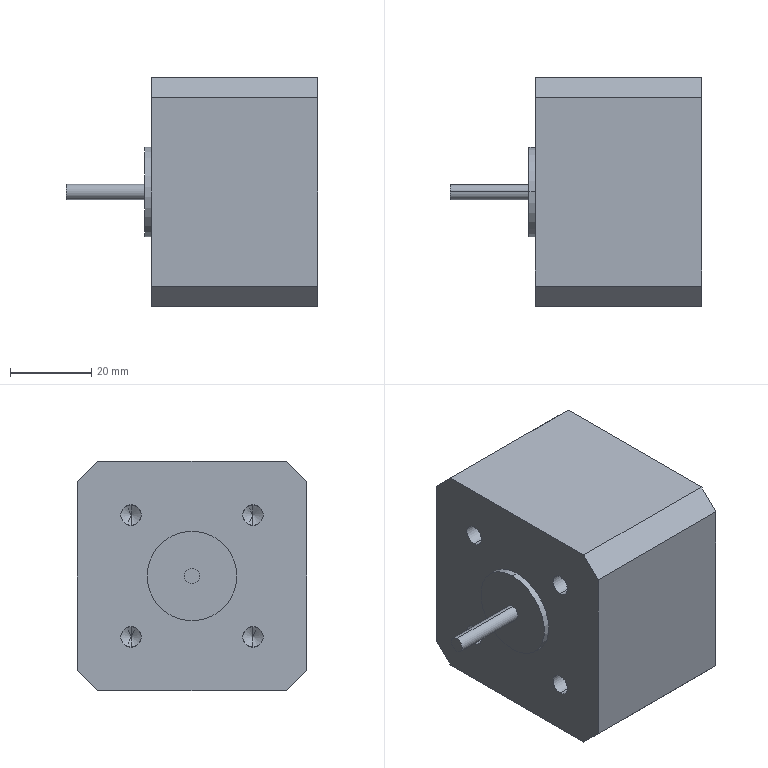Component | SolidWorks | 42StepperMotor-2 | 1 solid | 40 faces | box 62 x 56.4 x 56.4 mm | volume 128490 mm3 | cone 16 | cylinder 12 | plane 12 | commonest cylinder face diameters 5 x8 3.75 x2 22.1 x2
build123d program:
from build123d import *

# Parameters (mm, degrees)
BOSS_EXTRUDE1_DEPTH             = 41
SKETCH2_R                       = 11.05
BOSS_EXTRUDE2_DEPTH             = 1.6
SKETCH3_R                       = 1.875
BOSS_EXTRUDE3_DEPTH             = 19.4
F_5_0MM_DOWEL_HOLE1_D           = 5
F_5_0MM_DOWEL_HOLE1_DEPTH       = 8.5
F_5_0MM_DOWEL_HOLE1_CSINK_D     = 5.05
F_5_0MM_DOWEL_HOLE1_CSINK_ANGLE = 90
F_5_0MM_DOWEL_HOLE1_TIP         = 1.502


with BuildPart() as part:
    # Sketch1 → Boss-Extrude1 (new body)
    with BuildSketch(Plane.XY):
        Polygon((-28.2, 23.2), (-23.2, 28.2), (23.2, 28.2), (28.2, 23.2), (28.2, -23.2), (23.2, -28.2), (-23.2, -28.2), (-28.2, -23.2), align=None)
    extrude(amount=BOSS_EXTRUDE1_DEPTH)

    # Sketch2 → Boss-Extrude2 (add)
    with BuildSketch(Plane.XY.offset(41)):
        Circle(SKETCH2_R)
    extrude(amount=BOSS_EXTRUDE2_DEPTH)

    # Sketch3 → Boss-Extrude3 (add)
    with BuildSketch(Plane.XY.offset(42.6)):
        Circle(SKETCH3_R)
    extrude(amount=BOSS_EXTRUDE3_DEPTH)

    # 5.0mm Dowel Hole1
    with Locations(Plane.XY.offset(41)):
        with Locations((-15, 15), (15, 15), (-15, -15), (15, -15)):
            CounterSinkHole(F_5_0MM_DOWEL_HOLE1_D / 2, F_5_0MM_DOWEL_HOLE1_CSINK_D / 2, depth=F_5_0MM_DOWEL_HOLE1_DEPTH, counter_sink_angle=F_5_0MM_DOWEL_HOLE1_CSINK_ANGLE)
            with Locations((0, 0, -(F_5_0MM_DOWEL_HOLE1_DEPTH + F_5_0MM_DOWEL_HOLE1_TIP / 2))):  # 118° drill point
                Cone(0, F_5_0MM_DOWEL_HOLE1_D / 2, F_5_0MM_DOWEL_HOLE1_TIP, mode=Mode.SUBTRACT)


solid = part.part

# Placed as in the assembly
solid = solid.moved(Location((-67.419, 83, 36.5), (0, -90, 0)))
STEP:
#1=COLOUR_RGB('',0.7922,0.8196,0.9333);
#2=FILL_AREA_STYLE_COLOUR('',#1);
#3=FILL_AREA_STYLE('',(#2));
#4=SURFACE_STYLE_FILL_AREA(#3);
#5=SURFACE_SIDE_STYLE('',(#4));
#6=SURFACE_STYLE_USAGE(.BOTH.,#5);
#7=PRESENTATION_STYLE_ASSIGNMENT((#6));
#8=CARTESIAN_POINT('',(-4.267,3.858,0.748));
#9=VERTEX_POINT('',#8);
#10=CARTESIAN_POINT('',(-4.267,3.858,0.9449));
#11=VERTEX_POINT('',#10);
#12=CARTESIAN_POINT('',(-4.267,3.858,0.8465));
#13=DIRECTION('',(-1.,-0.,-0.));
#14=DIRECTION('',(0.,0.,1.));
#15=AXIS2_PLACEMENT_3D('',#12,#13,#14);
#16=CIRCLE('',#15,0.09843);
#17=EDGE_CURVE('',#9,#11,#16,.T.);
#18=ORIENTED_EDGE('',*,*,#17,.F.);
#19=CARTESIAN_POINT('',(-4.268,3.858,0.747));
#20=VERTEX_POINT('',#19);
#21=CARTESIAN_POINT('',(-4.268,3.858,0.747));
#22=DIRECTION('',(-0.7071,-0.,-0.7071));
#23=VECTOR('',#22,39.37);
#24=LINE('',#21,#23);
#25=EDGE_CURVE('',#9,#20,#24,.T.);
#26=ORIENTED_EDGE('',*,*,#25,.T.);
#27=CARTESIAN_POINT('',(-4.268,3.858,0.9459));
#28=VERTEX_POINT('',#27);
#29=CARTESIAN_POINT('',(-4.268,3.858,0.8465));
#30=DIRECTION('',(-1.,-0.,-0.));
#31=DIRECTION('',(0.,0.,1.));
#32=AXIS2_PLACEMENT_3D('',#29,#30,#31);
#33=CIRCLE('',#32,0.09941);
#34=EDGE_CURVE('',#20,#28,#33,.T.);
#35=ORIENTED_EDGE('',*,*,#34,.T.);
#36=CARTESIAN_POINT('',(-4.268,3.858,0.9459));
#37=DIRECTION('',(-0.7071,-0.,0.7071));
#38=VECTOR('',#37,39.37);
#39=LINE('',#36,#38);
#40=EDGE_CURVE('',#11,#28,#39,.T.);
#41=ORIENTED_EDGE('',*,*,#40,.F.);
#42=EDGE_LOOP('',(#18,#26,#35,#41));
#43=FACE_OUTER_BOUND('',#42,.T.);
#44=CARTESIAN_POINT('',(-4.268,3.858,0.8465));
#45=DIRECTION('',(-1.,-0.,-0.));
#46=DIRECTION('',(0.,0.,1.));
#47=AXIS2_PLACEMENT_3D('',#44,#45,#46);
#48=CONICAL_SURFACE('',#47,0.09941,0.7854);
#49=ADVANCED_FACE('',(#43),#48,.F.);
#50=CARTESIAN_POINT('',(-3.934,3.858,0.748));
#51=VERTEX_POINT('',#50);
#52=CARTESIAN_POINT('',(-3.934,3.858,0.9449));
#53=VERTEX_POINT('',#52);
#54=CARTESIAN_POINT('',(-3.934,3.858,0.8465));
#55=DIRECTION('',(-1.,-0.,-0.));
#56=DIRECTION('',(0.,0.,1.));
#57=AXIS2_PLACEMENT_3D('',#54,#55,#56);
#58=CIRCLE('',#57,0.09843);
#59=EDGE_CURVE('',#51,#53,#58,.T.);
#60=ORIENTED_EDGE('',*,*,#59,.F.);
#61=CARTESIAN_POINT('',(-4.268,3.858,0.748));
#62=DIRECTION('',(-1.,-0.,-0.));
#63=VECTOR('',#62,39.37);
#64=LINE('',#61,#63);
#65=EDGE_CURVE('',#51,#9,#64,.T.);
#66=ORIENTED_EDGE('',*,*,#65,.T.);
#67=ORIENTED_EDGE('',*,*,#17,.T.);
#68=CARTESIAN_POINT('',(-4.268,3.858,0.9449));
#69=DIRECTION('',(-1.,-0.,-0.));
#70=VECTOR('',#69,39.37);
#71=LINE('',#68,#70);
#72=EDGE_CURVE('',#53,#11,#71,.T.);
#73=ORIENTED_EDGE('',*,*,#72,.F.);
#74=EDGE_LOOP('',(#60,#66,#67,#73));
#75=FACE_OUTER_BOUND('',#74,.T.);
#76=CARTESIAN_POINT('',(-4.268,3.858,0.8465));
#77=DIRECTION('',(-1.,-0.,-0.));
#78=DIRECTION('',(0.,0.,1.));
#79=AXIS2_PLACEMENT_3D('',#76,#77,#78);
#80=CYLINDRICAL_SURFACE('',#79,0.09843);
#81=ADVANCED_FACE('',(#75),#80,.F.);
#82=CARTESIAN_POINT('',(-3.875,3.858,0.8465));
#83=VERTEX_POINT('',#82);
#84=CARTESIAN_POINT('',(-3.934,3.858,0.9449));
#85=DIRECTION('',(-0.515,-0.,0.8572));
#86=VECTOR('',#85,39.37);
#87=LINE('',#84,#86);
#88=EDGE_CURVE('',#83,#53,#87,.T.);
#89=ORIENTED_EDGE('',*,*,#88,.F.);
#90=CARTESIAN_POINT('',(-3.934,3.858,0.748));
#91=DIRECTION('',(-0.515,-0.,-0.8572));
#92=VECTOR('',#91,39.37);
#93=LINE('',#90,#92);
#94=EDGE_CURVE('',#83,#51,#93,.T.);
#95=ORIENTED_EDGE('',*,*,#94,.T.);
#96=ORIENTED_EDGE('',*,*,#59,.T.);
#97=EDGE_LOOP('',(#89,#95,#96));
#98=FACE_OUTER_BOUND('',#97,.T.);
#99=CARTESIAN_POINT('',(-3.934,3.858,0.8465));
#100=DIRECTION('',(-1.,-0.,-0.));
#101=DIRECTION('',(0.,0.,1.));
#102=AXIS2_PLACEMENT_3D('',#99,#100,#101);
#103=CONICAL_SURFACE('',#102,0.09843,1.03);
#104=ADVANCED_FACE('',(#98),#103,.F.);
#105=CARTESIAN_POINT('',(-4.267,3.858,1.929));
#106=VERTEX_POINT('',#105);
#107=CARTESIAN_POINT('',(-4.267,3.858,2.126));
#108=VERTEX_POINT('',#107);
#109=CARTESIAN_POINT('',(-4.267,3.858,2.028));
#110=DIRECTION('',(-1.,-0.,-0.));
#111=DIRECTION('',(0.,0.,1.));
#112=AXIS2_PLACEMENT_3D('',#109,#110,#111);
#113=CIRCLE('',#112,0.09843);
#114=EDGE_CURVE('',#106,#108,#113,.T.);
#115=ORIENTED_EDGE('',*,*,#114,.F.);
#116=CARTESIAN_POINT('',(-4.268,3.858,1.928));
#117=VERTEX_POINT('',#116);
#118=CARTESIAN_POINT('',(-4.268,3.858,1.928));
#119=DIRECTION('',(-0.7071,-0.,-0.7071));
#120=VECTOR('',#119,39.37);
#121=LINE('',#118,#120);
#122=EDGE_CURVE('',#106,#117,#121,.T.);
#123=ORIENTED_EDGE('',*,*,#122,.T.);
#124=CARTESIAN_POINT('',(-4.268,3.858,2.127));
#125=VERTEX_POINT('',#124);
#126=CARTESIAN_POINT('',(-4.268,3.858,2.028));
#127=DIRECTION('',(-1.,-0.,-0.));
#128=DIRECTION('',(0.,0.,1.));
#129=AXIS2_PLACEMENT_3D('',#126,#127,#128);
#130=CIRCLE('',#129,0.09941);
#131=EDGE_CURVE('',#117,#125,#130,.T.);
#132=ORIENTED_EDGE('',*,*,#131,.T.);
#133=CARTESIAN_POINT('',(-4.268,3.858,2.127));
#134=DIRECTION('',(-0.7071,-0.,0.7071));
#135=VECTOR('',#134,39.37);
#136=LINE('',#133,#135);
#137=EDGE_CURVE('',#108,#125,#136,.T.);
#138=ORIENTED_EDGE('',*,*,#137,.F.);
#139=EDGE_LOOP('',(#115,#123,#132,#138));
#140=FACE_OUTER_BOUND('',#139,.T.);
#141=CARTESIAN_POINT('',(-4.268,3.858,2.028));
#142=DIRECTION('',(-1.,-0.,-0.));
#143=DIRECTION('',(0.,0.,1.));
#144=AXIS2_PLACEMENT_3D('',#141,#142,#143);
#145=CONICAL_SURFACE('',#144,0.09941,0.7854);
#146=ADVANCED_FACE('',(#140),#145,.F.);
#147=CARTESIAN_POINT('',(-3.934,3.858,1.929));
#148=VERTEX_POINT('',#147);
#149=CARTESIAN_POINT('',(-3.934,3.858,2.126));
#150=VERTEX_POINT('',#149);
#151=CARTESIAN_POINT('',(-3.934,3.858,2.028));
#152=DIRECTION('',(-1.,-0.,-0.));
#153=DIRECTION('',(0.,0.,1.));
#154=AXIS2_PLACEMENT_3D('',#151,#152,#153);
#155=CIRCLE('',#154,0.09843);
#156=EDGE_CURVE('',#148,#150,#155,.T.);
#157=ORIENTED_EDGE('',*,*,#156,.F.);
#158=CARTESIAN_POINT('',(-4.268,3.858,1.929));
#159=DIRECTION('',(-1.,-0.,-0.));
#160=VECTOR('',#159,39.37);
#161=LINE('',#158,#160);
#162=EDGE_CURVE('',#148,#106,#161,.T.);
#163=ORIENTED_EDGE('',*,*,#162,.T.);
#164=ORIENTED_EDGE('',*,*,#114,.T.);
#165=CARTESIAN_POINT('',(-4.268,3.858,2.126));
#166=DIRECTION('',(-1.,-0.,-0.));
#167=VECTOR('',#166,39.37);
#168=LINE('',#165,#167);
#169=EDGE_CURVE('',#150,#108,#168,.T.);
#170=ORIENTED_EDGE('',*,*,#169,.F.);
#171=EDGE_LOOP('',(#157,#163,#164,#170));
#172=FACE_OUTER_BOUND('',#171,.T.);
#173=CARTESIAN_POINT('',(-4.268,3.858,2.028));
#174=DIRECTION('',(-1.,-0.,-0.));
#175=DIRECTION('',(0.,0.,1.));
#176=AXIS2_PLACEMENT_3D('',#173,#174,#175);
#177=CYLINDRICAL_SURFACE('',#176,0.09843);
#178=ADVANCED_FACE('',(#172),#177,.F.);
#179=CARTESIAN_POINT('',(-3.875,3.858,2.028));
#180=VERTEX_POINT('',#179);
#181=CARTESIAN_POINT('',(-3.934,3.858,2.126));
#182=DIRECTION('',(-0.515,-0.,0.8572));
#183=VECTOR('',#182,39.37);
#184=LINE('',#181,#183);
#185=EDGE_CURVE('',#180,#150,#184,.T.);
#186=ORIENTED_EDGE('',*,*,#185,.F.);
#187=CARTESIAN_POINT('',(-3.934,3.858,1.929));
#188=DIRECTION('',(-0.515,-0.,-0.8572));
#189=VECTOR('',#188,39.37);
#190=LINE('',#187,#189);
#191=EDGE_CURVE('',#180,#148,#190,.T.);
#192=ORIENTED_EDGE('',*,*,#191,.T.);
#193=ORIENTED_EDGE('',*,*,#156,.T.);
#194=EDGE_LOOP('',(#186,#192,#193));
#195=FACE_OUTER_BOUND('',#194,.T.);
#196=CARTESIAN_POINT('',(-3.934,3.858,2.028));
#197=DIRECTION('',(-1.,-0.,-0.));
#198=DIRECTION('',(0.,0.,1.));
#199=AXIS2_PLACEMENT_3D('',#196,#197,#198);
#200=CONICAL_SURFACE('',#199,0.09843,1.03);
#201=ADVANCED_FACE('',(#195),#200,.F.);
#202=CARTESIAN_POINT('',(-4.267,2.677,0.748));
#203=VERTEX_POINT('',#202);
#204=CARTESIAN_POINT('',(-4.267,2.677,0.9449));
#205=VERTEX_POINT('',#204);
#206=CARTESIAN_POINT('',(-4.267,2.677,0.8465));
#207=DIRECTION('',(-1.,-0.,-0.));
#208=DIRECTION('',(0.,0.,1.));
#209=AXIS2_PLACEMENT_3D('',#206,#207,#208);
#210=CIRCLE('',#209,0.09843);
#211=EDGE_CURVE('',#203,#205,#210,.T.);
#212=ORIENTED_EDGE('',*,*,#211,.F.);
#213=CARTESIAN_POINT('',(-4.268,2.677,0.747));
#214=VERTEX_POINT('',#213);
#215=CARTESIAN_POINT('',(-4.268,2.677,0.747));
#216=DIRECTION('',(-0.7071,-0.,-0.7071));
#217=VECTOR('',#216,39.37);
#218=LINE('',#215,#217);
#219=EDGE_CURVE('',#203,#214,#218,.T.);
#220=ORIENTED_EDGE('',*,*,#219,.T.);
#221=CARTESIAN_POINT('',(-4.268,2.677,0.9459));
#222=VERTEX_POINT('',#221);
#223=CARTESIAN_POINT('',(-4.268,2.677,0.8465));
#224=DIRECTION('',(-1.,-0.,-0.));
#225=DIRECTION('',(0.,0.,1.));
#226=AXIS2_PLACEMENT_3D('',#223,#224,#225);
#227=CIRCLE('',#226,0.09941);
#228=EDGE_CURVE('',#214,#222,#227,.T.);
#229=ORIENTED_EDGE('',*,*,#228,.T.);
#230=CARTESIAN_POINT('',(-4.268,2.677,0.9459));
#231=DIRECTION('',(-0.7071,-0.,0.7071));
#232=VECTOR('',#231,39.37);
#233=LINE('',#230,#232);
#234=EDGE_CURVE('',#205,#222,#233,.T.);
#235=ORIENTED_EDGE('',*,*,#234,.F.);
#236=EDGE_LOOP('',(#212,#220,#229,#235));
#237=FACE_OUTER_BOUND('',#236,.T.);
#238=CARTESIAN_POINT('',(-4.268,2.677,0.8465));
#239=DIRECTION('',(-1.,-0.,-0.));
#240=DIRECTION('',(0.,0.,1.));
#241=AXIS2_PLACEMENT_3D('',#238,#239,#240);
#242=CONICAL_SURFACE('',#241,0.09941,0.7854);
#243=ADVANCED_FACE('',(#237),#242,.F.);
#244=CARTESIAN_POINT('',(-3.934,2.677,0.748));
#245=VERTEX_POINT('',#244);
#246=CARTESIAN_POINT('',(-3.934,2.677,0.9449));
#247=VERTEX_POINT('',#246);
#248=CARTESIAN_POINT('',(-3.934,2.677,0.8465));
#249=DIRECTION('',(-1.,-0.,-0.));
#250=DIRECTION('',(0.,0.,1.));
#251=AXIS2_PLACEMENT_3D('',#248,#249,#250);
#252=CIRCLE('',#251,0.09843);
#253=EDGE_CURVE('',#245,#247,#252,.T.);
#254=ORIENTED_EDGE('',*,*,#253,.F.);
#255=CARTESIAN_POINT('',(-4.268,2.677,0.748));
#256=DIRECTION('',(-1.,-0.,-0.));
#257=VECTOR('',#256,39.37);
#258=LINE('',#255,#257);
#259=EDGE_CURVE('',#245,#203,#258,.T.);
#260=ORIENTED_EDGE('',*,*,#259,.T.);
#261=ORIENTED_EDGE('',*,*,#211,.T.);
#262=CARTESIAN_POINT('',(-4.268,2.677,0.9449));
#263=DIRECTION('',(-1.,-0.,-0.));
#264=VECTOR('',#263,39.37);
#265=LINE('',#262,#264);
#266=EDGE_CURVE('',#247,#205,#265,.T.);
#267=ORIENTED_EDGE('',*,*,#266,.F.);
#268=EDGE_LOOP('',(#254,#260,#261,#267));
#269=FACE_OUTER_BOUND('',#268,.T.);
#270=CARTESIAN_POINT('',(-4.268,2.677,0.8465));
#271=DIRECTION('',(-1.,-0.,-0.));
#272=DIRECTION('',(0.,0.,1.));
#273=AXIS2_PLACEMENT_3D('',#270,#271,#272);
#274=CYLINDRICAL_SURFACE('',#273,0.09843);
#275=ADVANCED_FACE('',(#269),#274,.F.);
#276=CARTESIAN_POINT('',(-3.875,2.677,0.8465));
#277=VERTEX_POINT('',#276);
#278=CARTESIAN_POINT('',(-3.934,2.677,0.9449));
#279=DIRECTION('',(-0.515,-0.,0.8572));
#280=VECTOR('',#279,39.37);
#281=LINE('',#278,#280);
#282=EDGE_CURVE('',#277,#247,#281,.T.);
#283=ORIENTED_EDGE('',*,*,#282,.F.);
#284=CARTESIAN_POINT('',(-3.934,2.677,0.748));
#285=DIRECTION('',(-0.515,-0.,-0.8572));
#286=VECTOR('',#285,39.37);
#287=LINE('',#284,#286);
#288=EDGE_CURVE('',#277,#245,#287,.T.);
#289=ORIENTED_EDGE('',*,*,#288,.T.);
#290=ORIENTED_EDGE('',*,*,#253,.T.);
#291=EDGE_LOOP('',(#283,#289,#290));
#292=FACE_OUTER_BOUND('',#291,.T.);
#293=CARTESIAN_POINT('',(-3.934,2.677,0.8465));
#294=DIRECTION('',(-1.,-0.,-0.));
#295=DIRECTION('',(0.,0.,1.));
#296=AXIS2_PLACEMENT_3D('',#293,#294,#295);
#297=CONICAL_SURFACE('',#296,0.09843,1.03);
#298=ADVANCED_FACE('',(#292),#297,.F.);
#299=CARTESIAN_POINT('',(-4.267,2.677,1.929));
#300=VERTEX_POINT('',#299);
#301=CARTESIAN_POINT('',(-4.267,2.677,2.126));
#302=VERTEX_POINT('',#301);
#303=CARTESIAN_POINT('',(-4.267,2.677,2.028));
#304=DIRECTION('',(-1.,-0.,-0.));
#305=DIRECTION('',(0.,0.,1.));
#306=AXIS2_PLACEMENT_3D('',#303,#304,#305);
#307=CIRCLE('',#306,0.09843);
#308=EDGE_CURVE('',#300,#302,#307,.T.);
#309=ORIENTED_EDGE('',*,*,#308,.F.);
#310=CARTESIAN_POINT('',(-4.268,2.677,1.928));
#311=VERTEX_POINT('',#310);
#312=CARTESIAN_POINT('',(-4.268,2.677,1.928));
#313=DIRECTION('',(-0.7071,-0.,-0.7071));
#314=VECTOR('',#313,39.37);
#315=LINE('',#312,#314);
#316=EDGE_CURVE('',#300,#311,#315,.T.);
#317=ORIENTED_EDGE('',*,*,#316,.T.);
#318=CARTESIAN_POINT('',(-4.268,2.677,2.127));
#319=VERTEX_POINT('',#318);
#320=CARTESIAN_POINT('',(-4.268,2.677,2.028));
#321=DIRECTION('',(-1.,-0.,-0.));
#322=DIRECTION('',(0.,0.,1.));
#323=AXIS2_PLACEMENT_3D('',#320,#321,#322);
#324=CIRCLE('',#323,0.09941);
#325=EDGE_CURVE('',#311,#319,#324,.T.);
#326=ORIENTED_EDGE('',*,*,#325,.T.);
#327=CARTESIAN_POINT('',(-4.268,2.677,2.127));
#328=DIRECTION('',(-0.7071,-0.,0.7071));
#329=VECTOR('',#328,39.37);
#330=LINE('',#327,#329);
#331=EDGE_CURVE('',#302,#319,#330,.T.);
#332=ORIENTED_EDGE('',*,*,#331,.F.);
#333=EDGE_LOOP('',(#309,#317,#326,#332));
#334=FACE_OUTER_BOUND('',#333,.T.);
#335=CARTESIAN_POINT('',(-4.268,2.677,2.028));
#336=DIRECTION('',(-1.,-0.,-0.));
#337=DIRECTION('',(0.,0.,1.));
#338=AXIS2_PLACEMENT_3D('',#335,#336,#337);
#339=CONICAL_SURFACE('',#338,0.09941,0.7854);
#340=ADVANCED_FACE('',(#334),#339,.F.);
#341=CARTESIAN_POINT('',(-3.934,2.677,1.929));
#342=VERTEX_POINT('',#341);
#343=CARTESIAN_POINT('',(-3.934,2.677,2.126));
#344=VERTEX_POINT('',#343);
#345=CARTESIAN_POINT('',(-3.934,2.677,2.028));
#346=DIRECTION('',(-1.,-0.,-0.));
#347=DIRECTION('',(0.,0.,1.));
#348=AXIS2_PLACEMENT_3D('',#345,#346,#347);
#349=CIRCLE('',#348,0.09843);
#350=EDGE_CURVE('',#342,#344,#349,.T.);
#351=ORIENTED_EDGE('',*,*,#350,.F.);
#352=CARTESIAN_POINT('',(-4.268,2.677,1.929));
#353=DIRECTION('',(-1.,-0.,-0.));
#354=VECTOR('',#353,39.37);
#355=LINE('',#352,#354);
#356=EDGE_CURVE('',#342,#300,#355,.T.);
#357=ORIENTED_EDGE('',*,*,#356,.T.);
#358=ORIENTED_EDGE('',*,*,#308,.T.);
#359=CARTESIAN_POINT('',(-4.268,2.677,2.126));
#360=DIRECTION('',(-1.,-0.,-0.));
#361=VECTOR('',#360,39.37);
#362=LINE('',#359,#361);
#363=EDGE_CURVE('',#344,#302,#362,.T.);
#364=ORIENTED_EDGE('',*,*,#363,.F.);
#365=EDGE_LOOP('',(#351,#357,#358,#364));
#366=FACE_OUTER_BOUND('',#365,.T.);
#367=CARTESIAN_POINT('',(-4.268,2.677,2.028));
#368=DIRECTION('',(-1.,-0.,-0.));
#369=DIRECTION('',(0.,0.,1.));
#370=AXIS2_PLACEMENT_3D('',#367,#368,#369);
#371=CYLINDRICAL_SURFACE('',#370,0.09843);
#372=ADVANCED_FACE('',(#366),#371,.F.);
#373=CARTESIAN_POINT('',(-3.875,2.677,2.028));
#374=VERTEX_POINT('',#373);
#375=CARTESIAN_POINT('',(-3.934,2.677,2.126));
#376=DIRECTION('',(-0.515,-0.,0.8572));
#377=VECTOR('',#376,39.37);
#378=LINE('',#375,#377);
#379=EDGE_CURVE('',#374,#344,#378,.T.);
#380=ORIENTED_EDGE('',*,*,#379,.F.);
#381=CARTESIAN_POINT('',(-3.934,2.677,1.929));
#382=DIRECTION('',(-0.515,-0.,-0.8572));
#383=VECTOR('',#382,39.37);
#384=LINE('',#381,#383);
#385=EDGE_CURVE('',#374,#342,#384,.T.);
#386=ORIENTED_EDGE('',*,*,#385,.T.);
#387=ORIENTED_EDGE('',*,*,#350,.T.);
#388=EDGE_LOOP('',(#380,#386,#387));
#389=FACE_OUTER_BOUND('',#388,.T.);
#390=CARTESIAN_POINT('',(-3.934,2.677,2.028));
#391=DIRECTION('',(-1.,-0.,-0.));
#392=DIRECTION('',(0.,0.,1.));
#393=AXIS2_PLACEMENT_3D('',#390,#391,#392);
#394=CONICAL_SURFACE('',#393,0.09843,1.03);
#395=ADVANCED_FACE('',(#389),#394,.F.);
#396=CARTESIAN_POINT('',(-5.095,3.268,1.511));
#397=VERTEX_POINT('',#396);
#398=CARTESIAN_POINT('',(-5.095,3.268,1.363));
#399=VERTEX_POINT('',#398);
#400=CARTESIAN_POINT('',(-5.095,3.268,1.437));
#401=DIRECTION('',(-1.,-0.,-0.));
#402=DIRECTION('',(0.,0.,1.));
#403=AXIS2_PLACEMENT_3D('',#400,#401,#402);
#404=CIRCLE('',#403,0.07382);
#405=EDGE_CURVE('',#397,#399,#404,.T.);
#406=ORIENTED_EDGE('',*,*,#405,.F.);
#407=CARTESIAN_POINT('',(-4.331,3.268,1.511));
#408=VERTEX_POINT('',#407);
#409=CARTESIAN_POINT('',(-5.095,3.268,1.511));
#410=DIRECTION('',(1.,0.,0.));
#411=VECTOR('',#410,39.37);
#412=LINE('',#409,#411);
#413=EDGE_CURVE('',#397,#408,#412,.T.);
#414=ORIENTED_EDGE('',*,*,#413,.T.);
#415=CARTESIAN_POINT('',(-4.331,3.268,1.363));
#416=VERTEX_POINT('',#415);
#417=CARTESIAN_POINT('',(-4.331,3.268,1.437));
#418=DIRECTION('',(-1.,-0.,-0.));
#419=DIRECTION('',(0.,0.,1.));
#420=AXIS2_PLACEMENT_3D('',#417,#418,#419);
#421=CIRCLE('',#420,0.07382);
#422=EDGE_CURVE('',#408,#416,#421,.T.);
#423=ORIENTED_EDGE('',*,*,#422,.T.);
#424=CARTESIAN_POINT('',(-5.095,3.268,1.363));
#425=DIRECTION('',(1.,0.,0.));
#426=VECTOR('',#425,39.37);
#427=LINE('',#424,#426);
#428=EDGE_CURVE('',#399,#416,#427,.T.);
#429=ORIENTED_EDGE('',*,*,#428,.F.);
#430=EDGE_LOOP('',(#406,#414,#423,#429));
#431=FACE_OUTER_BOUND('',#430,.T.);
#432=CARTESIAN_POINT('',(-5.095,3.268,1.437));
#433=DIRECTION('',(1.,0.,0.));
#434=DIRECTION('',(0.,0.,-1.));
#435=AXIS2_PLACEMENT_3D('',#432,#433,#434);
#436=CYLINDRICAL_SURFACE('',#435,0.07382);
#437=ADVANCED_FACE('',(#431),#436,.T.);
#438=CARTESIAN_POINT('',(-4.331,3.268,1.872));
#439=VERTEX_POINT('',#438);
#440=CARTESIAN_POINT('',(-4.331,3.268,1.002));
#441=VERTEX_POINT('',#440);
#442=CARTESIAN_POINT('',(-4.331,3.268,1.437));
#443=DIRECTION('',(-1.,-0.,-0.));
#444=DIRECTION('',(0.,0.,1.));
#445=AXIS2_PLACEMENT_3D('',#442,#443,#444);
#446=CIRCLE('',#445,0.435);
#447=EDGE_CURVE('',#439,#441,#446,.T.);
#448=ORIENTED_EDGE('',*,*,#447,.F.);
#449=CARTESIAN_POINT('',(-4.268,3.268,1.872));
#450=VERTEX_POINT('',#449);
#451=CARTESIAN_POINT('',(-4.331,3.268,1.872));
#452=DIRECTION('',(1.,0.,0.));
#453=VECTOR('',#452,39.37);
#454=LINE('',#451,#453);
#455=EDGE_CURVE('',#439,#450,#454,.T.);
#456=ORIENTED_EDGE('',*,*,#455,.T.);
#457=CARTESIAN_POINT('',(-4.268,3.268,1.002));
#458=VERTEX_POINT('',#457);
#459=CARTESIAN_POINT('',(-4.268,3.268,1.437));
#460=DIRECTION('',(-1.,-0.,-0.));
#461=DIRECTION('',(0.,0.,1.));
#462=AXIS2_PLACEMENT_3D('',#459,#460,#461);
#463=CIRCLE('',#462,0.435);
#464=EDGE_CURVE('',#450,#458,#463,.T.);
#465=ORIENTED_EDGE('',*,*,#464,.T.);
#466=CARTESIAN_POINT('',(-4.331,3.268,1.002));
#467=DIRECTION('',(1.,0.,0.));
#468=VECTOR('',#467,39.37);
#469=LINE('',#466,#468);
#470=EDGE_CURVE('',#441,#458,#469,.T.);
#471=ORIENTED_EDGE('',*,*,#470,.F.);
#472=EDGE_LOOP('',(#448,#456,#465,#471));
#473=FACE_OUTER_BOUND('',#472,.T.);
#474=CARTESIAN_POINT('',(-4.331,3.268,1.437));
#475=DIRECTION('',(1.,0.,0.));
#476=DIRECTION('',(0.,0.,-1.));
#477=AXIS2_PLACEMENT_3D('',#474,#475,#476);
#478=CYLINDRICAL_SURFACE('',#477,0.435);
#479=ADVANCED_FACE('',(#473),#478,.T.);
#480=CARTESIAN_POINT('',(-2.654,4.378,2.35));
#481=VERTEX_POINT('',#480);
#482=CARTESIAN_POINT('',(-2.654,4.378,0.5236));
#483=VERTEX_POINT('',#482);
#484=CARTESIAN_POINT('',(-2.654,4.378,0.5236));
#485=DIRECTION('',(0.,0.,-1.));
#486=VECTOR('',#485,39.37);
#487=LINE('',#484,#486);
#488=EDGE_CURVE('',#481,#483,#487,.T.);
#489=ORIENTED_EDGE('',*,*,#488,.T.);
#490=CARTESIAN_POINT('',(-4.268,4.378,0.5236));
#491=VERTEX_POINT('',#490);
#492=CARTESIAN_POINT('',(-4.268,4.378,0.5236));
#493=DIRECTION('',(1.,0.,0.));
#494=VECTOR('',#493,39.37);
#495=LINE('',#492,#494);
#496=EDGE_CURVE('',#491,#483,#495,.T.);
#497=ORIENTED_EDGE('',*,*,#496,.F.);
#498=CARTESIAN_POINT('',(-4.268,4.378,2.35));
#499=VERTEX_POINT('',#498);
#500=CARTESIAN_POINT('',(-4.268,4.378,0.5236));
#501=DIRECTION('',(0.,0.,-1.));
#502=VECTOR('',#501,39.37);
#503=LINE('',#500,#502);
#504=EDGE_CURVE('',#499,#491,#503,.T.);
#505=ORIENTED_EDGE('',*,*,#504,.F.);
#506=CARTESIAN_POINT('',(-4.268,4.378,2.35));
#507=DIRECTION('',(1.,0.,0.));
#508=VECTOR('',#507,39.37);
#509=LINE('',#506,#508);
#510=EDGE_CURVE('',#499,#481,#509,.T.);
#511=ORIENTED_EDGE('',*,*,#510,.T.);
#512=EDGE_LOOP('',(#489,#497,#505,#511));
#513=FACE_OUTER_BOUND('',#512,.T.);
#514=CARTESIAN_POINT('',(-4.268,4.378,0.5236));
#515=DIRECTION('',(0.,-1.,-0.));
#516=DIRECTION('',(1.,0.,0.));
#517=AXIS2_PLACEMENT_3D('',#514,#515,#516);
#518=PLANE('',#517);
#519=ADVANCED_FACE('',(#513),#518,.F.);
#520=CARTESIAN_POINT('',(-2.654,4.181,0.3268));
#521=VERTEX_POINT('',#520);
#522=CARTESIAN_POINT('',(-2.654,4.181,0.3268));
#523=DIRECTION('',(0.,-0.7071,-0.7071));
#524=VECTOR('',#523,39.37);
#525=LINE('',#522,#524);
#526=EDGE_CURVE('',#483,#521,#525,.T.);
#527=ORIENTED_EDGE('',*,*,#526,.T.);
#528=CARTESIAN_POINT('',(-4.268,4.181,0.3268));
#529=VERTEX_POINT('',#528);
#530=CARTESIAN_POINT('',(-4.268,4.181,0.3268));
#531=DIRECTION('',(1.,0.,0.));
#532=VECTOR('',#531,39.37);
#533=LINE('',#530,#532);
#534=EDGE_CURVE('',#529,#521,#533,.T.);
#535=ORIENTED_EDGE('',*,*,#534,.F.);
#536=CARTESIAN_POINT('',(-4.268,4.181,0.3268));
#537=DIRECTION('',(0.,-0.7071,-0.7071));
#538=VECTOR('',#537,39.37);
#539=LINE('',#536,#538);
#540=EDGE_CURVE('',#491,#529,#539,.T.);
#541=ORIENTED_EDGE('',*,*,#540,.F.);
#542=ORIENTED_EDGE('',*,*,#496,.T.);
#543=EDGE_LOOP('',(#527,#535,#541,#542));
#544=FACE_OUTER_BOUND('',#543,.T.);
#545=CARTESIAN_POINT('',(-4.268,4.181,0.3268));
#546=DIRECTION('',(0.,-0.7071,0.7071));
#547=DIRECTION('',(-0.,0.7071,0.7071));
#548=AXIS2_PLACEMENT_3D('',#545,#546,#547);
#549=PLANE('',#548);
#550=ADVANCED_FACE('',(#544),#549,.F.);
#551=CARTESIAN_POINT('',(-2.654,2.354,0.3268));
#552=VERTEX_POINT('',#551);
#553=CARTESIAN_POINT('',(-2.654,2.354,0.3268));
#554=DIRECTION('',(0.,-1.,-0.));
#555=VECTOR('',#554,39.37);
#556=LINE('',#553,#555);
#557=EDGE_CURVE('',#521,#552,#556,.T.);
#558=ORIENTED_EDGE('',*,*,#557,.T.);
#559=CARTESIAN_POINT('',(-4.268,2.354,0.3268));
#560=VERTEX_POINT('',#559);
#561=CARTESIAN_POINT('',(-4.268,2.354,0.3268));
#562=DIRECTION('',(1.,0.,0.));
#563=VECTOR('',#562,39.37);
#564=LINE('',#561,#563);
#565=EDGE_CURVE('',#560,#552,#564,.T.);
#566=ORIENTED_EDGE('',*,*,#565,.F.);
#567=CARTESIAN_POINT('',(-4.268,2.354,0.3268));
#568=DIRECTION('',(0.,-1.,-0.));
#569=VECTOR('',#568,39.37);
#570=LINE('',#567,#569);
#571=EDGE_CURVE('',#529,#560,#570,.T.);
#572=ORIENTED_EDGE('',*,*,#571,.F.);
#573=ORIENTED_EDGE('',*,*,#534,.T.);
#574=EDGE_LOOP('',(#558,#566,#572,#573));
#575=FACE_OUTER_BOUND('',#574,.T.);
#576=CARTESIAN_POINT('',(-4.268,2.354,0.3268));
#577=DIRECTION('',(-0.,-0.,1.));
#578=DIRECTION('',(-0.,1.,0.));
#579=AXIS2_PLACEMENT_3D('',#576,#577,#578);
#580=PLANE('',#579);
#581=ADVANCED_FACE('',(#575),#580,.F.);
#582=CARTESIAN_POINT('',(-2.654,2.157,0.5236));
#583=VERTEX_POINT('',#582);
#584=CARTESIAN_POINT('',(-2.654,2.354,0.3268));
#585=DIRECTION('',(0.,-0.7071,0.7071));
#586=VECTOR('',#585,39.37);
#587=LINE('',#584,#586);
#588=EDGE_CURVE('',#552,#583,#587,.T.);
#589=ORIENTED_EDGE('',*,*,#588,.T.);
#590=CARTESIAN_POINT('',(-4.268,2.157,0.5236));
#591=VERTEX_POINT('',#590);
#592=CARTESIAN_POINT('',(-4.268,2.157,0.5236));
#593=DIRECTION('',(1.,0.,0.));
#594=VECTOR('',#593,39.37);
#595=LINE('',#592,#594);
#596=EDGE_CURVE('',#591,#583,#595,.T.);
#597=ORIENTED_EDGE('',*,*,#596,.F.);
#598=CARTESIAN_POINT('',(-4.268,2.354,0.3268));
#599=DIRECTION('',(0.,-0.7071,0.7071));
#600=VECTOR('',#599,39.37);
#601=LINE('',#598,#600);
#602=EDGE_CURVE('',#560,#591,#601,.T.);
#603=ORIENTED_EDGE('',*,*,#602,.F.);
#604=ORIENTED_EDGE('',*,*,#565,.T.);
#605=EDGE_LOOP('',(#589,#597,#603,#604));
#606=FACE_OUTER_BOUND('',#605,.T.);
#607=CARTESIAN_POINT('',(-4.268,2.354,0.3268));
#608=DIRECTION('',(-0.,0.7071,0.7071));
#609=DIRECTION('',(-0.,0.7071,-0.7071));
#610=AXIS2_PLACEMENT_3D('',#607,#608,#609);
#611=PLANE('',#610);
#612=ADVANCED_FACE('',(#606),#611,.F.);
#613=CARTESIAN_POINT('',(-2.654,2.157,2.35));
#614=VERTEX_POINT('',#613);
#615=CARTESIAN_POINT('',(-2.654,2.157,0.5236));
#616=DIRECTION('',(-0.,-0.,1.));
#617=VECTOR('',#616,39.37);
#618=LINE('',#615,#617);
#619=EDGE_CURVE('',#583,#614,#618,.T.);
#620=ORIENTED_EDGE('',*,*,#619,.T.);
#621=CARTESIAN_POINT('',(-4.268,2.157,2.35));
#622=VERTEX_POINT('',#621);
#623=CARTESIAN_POINT('',(-4.268,2.157,2.35));
#624=DIRECTION('',(1.,0.,0.));
#625=VECTOR('',#624,39.37);
#626=LINE('',#623,#625);
#627=EDGE_CURVE('',#622,#614,#626,.T.);
#628=ORIENTED_EDGE('',*,*,#627,.F.);
#629=CARTESIAN_POINT('',(-4.268,2.157,0.5236));
#630=DIRECTION('',(-0.,-0.,1.));
#631=VECTOR('',#630,39.37);
#632=LINE('',#629,#631);
#633=EDGE_CURVE('',#591,#622,#632,.T.);
#634=ORIENTED_EDGE('',*,*,#633,.F.);
#635=ORIENTED_EDGE('',*,*,#596,.T.);
#636=EDGE_LOOP('',(#620,#628,#634,#635));
#637=FACE_OUTER_BOUND('',#636,.T.);
#638=CARTESIAN_POINT('',(-4.268,2.157,0.5236));
#639=DIRECTION('',(-0.,1.,0.));
#640=DIRECTION('',(-1.,-0.,-0.));
#641=AXIS2_PLACEMENT_3D('',#638,#639,#640);
#642=PLANE('',#641);
#643=ADVANCED_FACE('',(#637),#642,.F.);
#644=CARTESIAN_POINT('',(-2.654,2.354,2.547));
#645=VERTEX_POINT('',#644);
#646=CARTESIAN_POINT('',(-2.654,2.157,2.35));
#647=DIRECTION('',(-0.,0.7071,0.7071));
#648=VECTOR('',#647,39.37);
#649=LINE('',#646,#648);
#650=EDGE_CURVE('',#614,#645,#649,.T.);
#651=ORIENTED_EDGE('',*,*,#650,.T.);
#652=CARTESIAN_POINT('',(-4.268,2.354,2.547));
#653=VERTEX_POINT('',#652);
#654=CARTESIAN_POINT('',(-4.268,2.354,2.547));
#655=DIRECTION('',(1.,0.,0.));
#656=VECTOR('',#655,39.37);
#657=LINE('',#654,#656);
#658=EDGE_CURVE('',#653,#645,#657,.T.);
#659=ORIENTED_EDGE('',*,*,#658,.F.);
#660=CARTESIAN_POINT('',(-4.268,2.157,2.35));
#661=DIRECTION('',(-0.,0.7071,0.7071));
#662=VECTOR('',#661,39.37);
#663=LINE('',#660,#662);
#664=EDGE_CURVE('',#622,#653,#663,.T.);
#665=ORIENTED_EDGE('',*,*,#664,.F.);
#666=ORIENTED_EDGE('',*,*,#627,.T.);
#667=EDGE_LOOP('',(#651,#659,#665,#666));
#668=FACE_OUTER_BOUND('',#667,.T.);
#669=CARTESIAN_POINT('',(-4.268,2.157,2.35));
#670=DIRECTION('',(-0.,0.7071,-0.7071));
#671=DIRECTION('',(0.,-0.7071,-0.7071));
#672=AXIS2_PLACEMENT_3D('',#669,#670,#671);
#673=PLANE('',#672);
#674=ADVANCED_FACE('',(#668),#673,.F.);
#675=CARTESIAN_POINT('',(-2.654,4.181,2.547));
#676=VERTEX_POINT('',#675);
#677=CARTESIAN_POINT('',(-2.654,2.354,2.547));
#678=DIRECTION('',(-0.,1.,0.));
#679=VECTOR('',#678,39.37);
#680=LINE('',#677,#679);
#681=EDGE_CURVE('',#645,#676,#680,.T.);
#682=ORIENTED_EDGE('',*,*,#681,.T.);
#683=CARTESIAN_POINT('',(-4.268,4.181,2.547));
#684=VERTEX_POINT('',#683);
#685=CARTESIAN_POINT('',(-4.268,4.181,2.547));
#686=DIRECTION('',(1.,0.,0.));
#687=VECTOR('',#686,39.37);
#688=LINE('',#685,#687);
#689=EDGE_CURVE('',#684,#676,#688,.T.);
#690=ORIENTED_EDGE('',*,*,#689,.F.);
#691=CARTESIAN_POINT('',(-4.268,2.354,2.547));
#692=DIRECTION('',(-0.,1.,0.));
#693=VECTOR('',#692,39.37);
#694=LINE('',#691,#693);
#695=EDGE_CURVE('',#653,#684,#694,.T.);
#696=ORIENTED_EDGE('',*,*,#695,.F.);
#697=ORIENTED_EDGE('',*,*,#658,.T.);
#698=EDGE_LOOP('',(#682,#690,#696,#697));
#699=FACE_OUTER_BOUND('',#698,.T.);
#700=CARTESIAN_POINT('',(-4.268,2.354,2.547));
#701=DIRECTION('',(0.,0.,-1.));
#702=DIRECTION('',(-1.,-0.,-0.));
#703=AXIS2_PLACEMENT_3D('',#700,#701,#702);
#704=PLANE('',#703);
#705=ADVANCED_FACE('',(#699),#704,.F.);
#706=CARTESIAN_POINT('',(-2.654,4.181,2.547));
#707=DIRECTION('',(-0.,0.7071,-0.7071));
#708=VECTOR('',#707,39.37);
#709=LINE('',#706,#708);
#710=EDGE_CURVE('',#676,#481,#709,.T.);
#711=ORIENTED_EDGE('',*,*,#710,.T.);
#712=ORIENTED_EDGE('',*,*,#510,.F.);
#713=CARTESIAN_POINT('',(-4.268,4.181,2.547));
#714=DIRECTION('',(-0.,0.7071,-0.7071));
#715=VECTOR('',#714,39.37);
#716=LINE('',#713,#715);
#717=EDGE_CURVE('',#684,#499,#716,.T.);
#718=ORIENTED_EDGE('',*,*,#717,.F.);
#719=ORIENTED_EDGE('',*,*,#689,.T.);
#720=EDGE_LOOP('',(#711,#712,#718,#719));
#721=FACE_OUTER_BOUND('',#720,.T.);
#722=CARTESIAN_POINT('',(-4.268,4.181,2.547));
#723=DIRECTION('',(0.,-0.7071,-0.7071));
#724=DIRECTION('',(0.,-0.7071,0.7071));
#725=AXIS2_PLACEMENT_3D('',#722,#723,#724);
#726=PLANE('',#725);
#727=ADVANCED_FACE('',(#721),#726,.F.);
#728=CARTESIAN_POINT('',(-4.268,3.858,0.8465));
#729=DIRECTION('',(-1.,-0.,-0.));
#730=DIRECTION('',(0.,0.,1.));
#731=AXIS2_PLACEMENT_3D('',#728,#729,#730);
#732=CIRCLE('',#731,0.09941);
#733=EDGE_CURVE('',#28,#20,#732,.T.);
#734=ORIENTED_EDGE('',*,*,#733,.F.);
#735=ORIENTED_EDGE('',*,*,#34,.F.);
#736=EDGE_LOOP('',(#734,#735));
#737=FACE_BOUND('',#736,.T.);
#738=CARTESIAN_POINT('',(-4.268,3.858,2.028));
#739=DIRECTION('',(-1.,-0.,-0.));
#740=DIRECTION('',(0.,0.,1.));
#741=AXIS2_PLACEMENT_3D('',#738,#739,#740);
#742=CIRCLE('',#741,0.09941);
#743=EDGE_CURVE('',#125,#117,#742,.T.);
#744=ORIENTED_EDGE('',*,*,#743,.F.);
#745=ORIENTED_EDGE('',*,*,#131,.F.);
#746=EDGE_LOOP('',(#744,#745));
#747=FACE_BOUND('',#746,.T.);
#748=CARTESIAN_POINT('',(-4.268,2.677,0.8465));
#749=DIRECTION('',(-1.,-0.,-0.));
#750=DIRECTION('',(0.,0.,1.));
#751=AXIS2_PLACEMENT_3D('',#748,#749,#750);
#752=CIRCLE('',#751,0.09941);
#753=EDGE_CURVE('',#222,#214,#752,.T.);
#754=ORIENTED_EDGE('',*,*,#753,.F.);
#755=ORIENTED_EDGE('',*,*,#228,.F.);
#756=EDGE_LOOP('',(#754,#755));
#757=FACE_BOUND('',#756,.T.);
#758=CARTESIAN_POINT('',(-4.268,2.677,2.028));
#759=DIRECTION('',(-1.,-0.,-0.));
#760=DIRECTION('',(0.,0.,1.));
#761=AXIS2_PLACEMENT_3D('',#758,#759,#760);
#762=CIRCLE('',#761,0.09941);
#763=EDGE_CURVE('',#319,#311,#762,.T.);
#764=ORIENTED_EDGE('',*,*,#763,.F.);
#765=ORIENTED_EDGE('',*,*,#325,.F.);
#766=EDGE_LOOP('',(#764,#765));
#767=FACE_BOUND('',#766,.T.);
#768=CARTESIAN_POINT('',(-4.268,3.268,1.437));
#769=DIRECTION('',(-1.,-0.,-0.));
#770=DIRECTION('',(0.,0.,1.));
#771=AXIS2_PLACEMENT_3D('',#768,#769,#770);
#772=CIRCLE('',#771,0.435);
#773=EDGE_CURVE('',#458,#450,#772,.T.);
#774=ORIENTED_EDGE('',*,*,#773,.F.);
#775=ORIENTED_EDGE('',*,*,#464,.F.);
#776=EDGE_LOOP('',(#774,#775));
#777=FACE_BOUND('',#776,.T.);
#778=ORIENTED_EDGE('',*,*,#504,.T.);
#779=ORIENTED_EDGE('',*,*,#540,.T.);
#780=ORIENTED_EDGE('',*,*,#571,.T.);
#781=ORIENTED_EDGE('',*,*,#602,.T.);
#782=ORIENTED_EDGE('',*,*,#633,.T.);
#783=ORIENTED_EDGE('',*,*,#664,.T.);
#784=ORIENTED_EDGE('',*,*,#695,.T.);
#785=ORIENTED_EDGE('',*,*,#717,.T.);
#786=EDGE_LOOP('',(#778,#779,#780,#781,#782,#783,#784,#785));
#787=FACE_OUTER_BOUND('',#786,.T.);
#788=CARTESIAN_POINT('',(-4.268,3.268,1.437));
#789=DIRECTION('',(-1.,-0.,-0.));
#790=DIRECTION('',(-0.,-0.,1.));
#791=AXIS2_PLACEMENT_3D('',#788,#789,#790);
#792=PLANE('',#791);
#793=ADVANCED_FACE('',(#737,#747,#757,#767,#777,#787),#792,.T.);
#794=ORIENTED_EDGE('',*,*,#488,.F.);
#795=ORIENTED_EDGE('',*,*,#710,.F.);
#796=ORIENTED_EDGE('',*,*,#681,.F.);
#797=ORIENTED_EDGE('',*,*,#650,.F.);
#798=ORIENTED_EDGE('',*,*,#619,.F.);
#799=ORIENTED_EDGE('',*,*,#588,.F.);
#800=ORIENTED_EDGE('',*,*,#557,.F.);
#801=ORIENTED_EDGE('',*,*,#526,.F.);
#802=EDGE_LOOP('',(#794,#795,#796,#797,#798,#799,#800,#801));
#803=FACE_OUTER_BOUND('',#802,.T.);
#804=CARTESIAN_POINT('',(-2.654,3.268,1.437));
#805=DIRECTION('',(-1.,-0.,-0.));
#806=DIRECTION('',(-0.,-0.,1.));
#807=AXIS2_PLACEMENT_3D('',#804,#805,#806);
#808=PLANE('',#807);
#809=ADVANCED_FACE('',(#803),#808,.F.);
#810=ORIENTED_EDGE('',*,*,#455,.F.);
#811=CARTESIAN_POINT('',(-4.331,3.268,1.437));
#812=DIRECTION('',(-1.,-0.,-0.));
#813=DIRECTION('',(0.,0.,1.));
#814=AXIS2_PLACEMENT_3D('',#811,#812,#813);
#815=CIRCLE('',#814,0.435);
#816=EDGE_CURVE('',#441,#439,#815,.T.);
#817=ORIENTED_EDGE('',*,*,#816,.F.);
#818=ORIENTED_EDGE('',*,*,#470,.T.);
#819=ORIENTED_EDGE('',*,*,#773,.T.);
#820=EDGE_LOOP('',(#810,#817,#818,#819));
#821=FACE_OUTER_BOUND('',#820,.T.);
#822=CARTESIAN_POINT('',(-4.331,3.268,1.437));
#823=DIRECTION('',(1.,0.,0.));
#824=DIRECTION('',(0.,0.,-1.));
#825=AXIS2_PLACEMENT_3D('',#822,#823,#824);
#826=CYLINDRICAL_SURFACE('',#825,0.435);
#827=ADVANCED_FACE('',(#821),#826,.T.);
#828=CARTESIAN_POINT('',(-4.331,3.268,1.437));
#829=DIRECTION('',(-1.,-0.,-0.));
#830=DIRECTION('',(0.,0.,1.));
#831=AXIS2_PLACEMENT_3D('',#828,#829,#830);
#832=CIRCLE('',#831,0.07382);
#833=EDGE_CURVE('',#416,#408,#832,.T.);
#834=ORIENTED_EDGE('',*,*,#833,.F.);
#835=ORIENTED_EDGE('',*,*,#422,.F.);
#836=EDGE_LOOP('',(#834,#835));
#837=FACE_BOUND('',#836,.T.);
#838=ORIENTED_EDGE('',*,*,#816,.T.);
#839=ORIENTED_EDGE('',*,*,#447,.T.);
#840=EDGE_LOOP('',(#838,#839));
#841=FACE_OUTER_BOUND('',#840,.T.);
#842=CARTESIAN_POINT('',(-4.331,3.268,1.437));
#843=DIRECTION('',(-1.,-0.,-0.));
#844=DIRECTION('',(-0.,-0.,1.));
#845=AXIS2_PLACEMENT_3D('',#842,#843,#844);
#846=PLANE('',#845);
#847=ADVANCED_FACE('',(#837,#841),#846,.T.);
#848=ORIENTED_EDGE('',*,*,#413,.F.);
#849=CARTESIAN_POINT('',(-5.095,3.268,1.437));
#850=DIRECTION('',(-1.,-0.,-0.));
#851=DIRECTION('',(0.,0.,1.));
#852=AXIS2_PLACEMENT_3D('',#849,#850,#851);
#853=CIRCLE('',#852,0.07382);
#854=EDGE_CURVE('',#399,#397,#853,.T.);
#855=ORIENTED_EDGE('',*,*,#854,.F.);
#856=ORIENTED_EDGE('',*,*,#428,.T.);
#857=ORIENTED_EDGE('',*,*,#833,.T.);
#858=EDGE_LOOP('',(#848,#855,#856,#857));
#859=FACE_OUTER_BOUND('',#858,.T.);
#860=CARTESIAN_POINT('',(-5.095,3.268,1.437));
#861=DIRECTION('',(1.,0.,0.));
#862=DIRECTION('',(0.,0.,-1.));
#863=AXIS2_PLACEMENT_3D('',#860,#861,#862);
#864=CYLINDRICAL_SURFACE('',#863,0.07382);
#865=ADVANCED_FACE('',(#859),#864,.T.);
#866=ORIENTED_EDGE('',*,*,#854,.T.);
#867=ORIENTED_EDGE('',*,*,#405,.T.);
#868=EDGE_LOOP('',(#866,#867));
#869=FACE_OUTER_BOUND('',#868,.T.);
#870=CARTESIAN_POINT('',(-5.095,3.268,1.437));
#871=DIRECTION('',(-1.,-0.,-0.));
#872=DIRECTION('',(-0.,-0.,1.));
#873=AXIS2_PLACEMENT_3D('',#870,#871,#872);
#874=PLANE('',#873);
#875=ADVANCED_FACE('',(#869),#874,.T.);
#876=ORIENTED_EDGE('',*,*,#385,.F.);
#877=ORIENTED_EDGE('',*,*,#379,.T.);
#878=CARTESIAN_POINT('',(-3.934,2.677,2.028));
#879=DIRECTION('',(-1.,-0.,-0.));
#880=DIRECTION('',(0.,0.,1.));
#881=AXIS2_PLACEMENT_3D('',#878,#879,#880);
#882=CIRCLE('',#881,0.09843);
#883=EDGE_CURVE('',#344,#342,#882,.T.);
#884=ORIENTED_EDGE('',*,*,#883,.T.);
#885=EDGE_LOOP('',(#876,#877,#884));
#886=FACE_OUTER_BOUND('',#885,.T.);
#887=CARTESIAN_POINT('',(-3.934,2.677,2.028));
#888=DIRECTION('',(-1.,-0.,-0.));
#889=DIRECTION('',(0.,0.,1.));
#890=AXIS2_PLACEMENT_3D('',#887,#888,#889);
#891=CONICAL_SURFACE('',#890,0.09843,1.03);
#892=ADVANCED_FACE('',(#886),#891,.F.);
#893=ORIENTED_EDGE('',*,*,#356,.F.);
#894=ORIENTED_EDGE('',*,*,#883,.F.);
#895=ORIENTED_EDGE('',*,*,#363,.T.);
#896=CARTESIAN_POINT('',(-4.267,2.677,2.028));
#897=DIRECTION('',(-1.,-0.,-0.));
#898=DIRECTION('',(0.,0.,1.));
#899=AXIS2_PLACEMENT_3D('',#896,#897,#898);
#900=CIRCLE('',#899,0.09843);
#901=EDGE_CURVE('',#302,#300,#900,.T.);
#902=ORIENTED_EDGE('',*,*,#901,.T.);
#903=EDGE_LOOP('',(#893,#894,#895,#902));
#904=FACE_OUTER_BOUND('',#903,.T.);
#905=CARTESIAN_POINT('',(-4.268,2.677,2.028));
#906=DIRECTION('',(-1.,-0.,-0.));
#907=DIRECTION('',(0.,0.,1.));
#908=AXIS2_PLACEMENT_3D('',#905,#906,#907);
#909=CYLINDRICAL_SURFACE('',#908,0.09843);
#910=ADVANCED_FACE('',(#904),#909,.F.);
#911=ORIENTED_EDGE('',*,*,#316,.F.);
#912=ORIENTED_EDGE('',*,*,#901,.F.);
#913=ORIENTED_EDGE('',*,*,#331,.T.);
#914=ORIENTED_EDGE('',*,*,#763,.T.);
#915=EDGE_LOOP('',(#911,#912,#913,#914));
#916=FACE_OUTER_BOUND('',#915,.T.);
#917=CARTESIAN_POINT('',(-4.268,2.677,2.028));
#918=DIRECTION('',(-1.,-0.,-0.));
#919=DIRECTION('',(0.,0.,1.));
#920=AXIS2_PLACEMENT_3D('',#917,#918,#919);
#921=CONICAL_SURFACE('',#920,0.09941,0.7854);
#922=ADVANCED_FACE('',(#916),#921,.F.);
#923=ORIENTED_EDGE('',*,*,#288,.F.);
#924=ORIENTED_EDGE('',*,*,#282,.T.);
#925=CARTESIAN_POINT('',(-3.934,2.677,0.8465));
#926=DIRECTION('',(-1.,-0.,-0.));
#927=DIRECTION('',(0.,0.,1.));
#928=AXIS2_PLACEMENT_3D('',#925,#926,#927);
#929=CIRCLE('',#928,0.09843);
#930=EDGE_CURVE('',#247,#245,#929,.T.);
#931=ORIENTED_EDGE('',*,*,#930,.T.);
#932=EDGE_LOOP('',(#923,#924,#931));
#933=FACE_OUTER_BOUND('',#932,.T.);
#934=CARTESIAN_POINT('',(-3.934,2.677,0.8465));
#935=DIRECTION('',(-1.,-0.,-0.));
#936=DIRECTION('',(0.,0.,1.));
#937=AXIS2_PLACEMENT_3D('',#934,#935,#936);
#938=CONICAL_SURFACE('',#937,0.09843,1.03);
#939=ADVANCED_FACE('',(#933),#938,.F.);
#940=ORIENTED_EDGE('',*,*,#259,.F.);
#941=ORIENTED_EDGE('',*,*,#930,.F.);
#942=ORIENTED_EDGE('',*,*,#266,.T.);
#943=CARTESIAN_POINT('',(-4.267,2.677,0.8465));
#944=DIRECTION('',(-1.,-0.,-0.));
#945=DIRECTION('',(0.,0.,1.));
#946=AXIS2_PLACEMENT_3D('',#943,#944,#945);
#947=CIRCLE('',#946,0.09843);
#948=EDGE_CURVE('',#205,#203,#947,.T.);
#949=ORIENTED_EDGE('',*,*,#948,.T.);
#950=EDGE_LOOP('',(#940,#941,#942,#949));
#951=FACE_OUTER_BOUND('',#950,.T.);
#952=CARTESIAN_POINT('',(-4.268,2.677,0.8465));
#953=DIRECTION('',(-1.,-0.,-0.));
#954=DIRECTION('',(0.,0.,1.));
#955=AXIS2_PLACEMENT_3D('',#952,#953,#954);
#956=CYLINDRICAL_SURFACE('',#955,0.09843);
#957=ADVANCED_FACE('',(#951),#956,.F.);
#958=ORIENTED_EDGE('',*,*,#219,.F.);
#959=ORIENTED_EDGE('',*,*,#948,.F.);
#960=ORIENTED_EDGE('',*,*,#234,.T.);
#961=ORIENTED_EDGE('',*,*,#753,.T.);
#962=EDGE_LOOP('',(#958,#959,#960,#961));
#963=FACE_OUTER_BOUND('',#962,.T.);
#964=CARTESIAN_POINT('',(-4.268,2.677,0.8465));
#965=DIRECTION('',(-1.,-0.,-0.));
#966=DIRECTION('',(0.,0.,1.));
#967=AXIS2_PLACEMENT_3D('',#964,#965,#966);
#968=CONICAL_SURFACE('',#967,0.09941,0.7854);
#969=ADVANCED_FACE('',(#963),#968,.F.);
#970=ORIENTED_EDGE('',*,*,#191,.F.);
#971=ORIENTED_EDGE('',*,*,#185,.T.);
#972=CARTESIAN_POINT('',(-3.934,3.858,2.028));
#973=DIRECTION('',(-1.,-0.,-0.));
#974=DIRECTION('',(0.,0.,1.));
#975=AXIS2_PLACEMENT_3D('',#972,#973,#974);
#976=CIRCLE('',#975,0.09843);
#977=EDGE_CURVE('',#150,#148,#976,.T.);
#978=ORIENTED_EDGE('',*,*,#977,.T.);
#979=EDGE_LOOP('',(#970,#971,#978));
#980=FACE_OUTER_BOUND('',#979,.T.);
#981=CARTESIAN_POINT('',(-3.934,3.858,2.028));
#982=DIRECTION('',(-1.,-0.,-0.));
#983=DIRECTION('',(0.,0.,1.));
#984=AXIS2_PLACEMENT_3D('',#981,#982,#983);
#985=CONICAL_SURFACE('',#984,0.09843,1.03);
#986=ADVANCED_FACE('',(#980),#985,.F.);
#987=ORIENTED_EDGE('',*,*,#162,.F.);
#988=ORIENTED_EDGE('',*,*,#977,.F.);
#989=ORIENTED_EDGE('',*,*,#169,.T.);
#990=CARTESIAN_POINT('',(-4.267,3.858,2.028));
#991=DIRECTION('',(-1.,-0.,-0.));
#992=DIRECTION('',(0.,0.,1.));
#993=AXIS2_PLACEMENT_3D('',#990,#991,#992);
#994=CIRCLE('',#993,0.09843);
#995=EDGE_CURVE('',#108,#106,#994,.T.);
#996=ORIENTED_EDGE('',*,*,#995,.T.);
#997=EDGE_LOOP('',(#987,#988,#989,#996));
#998=FACE_OUTER_BOUND('',#997,.T.);
#999=CARTESIAN_POINT('',(-4.268,3.858,2.028));
#1000=DIRECTION('',(-1.,-0.,-0.));
#1001=DIRECTION('',(0.,0.,1.));
#1002=AXIS2_PLACEMENT_3D('',#999,#1000,#1001);
#1003=CYLINDRICAL_SURFACE('',#1002,0.09843);
#1004=ADVANCED_FACE('',(#998),#1003,.F.);
#1005=ORIENTED_EDGE('',*,*,#122,.F.);
#1006=ORIENTED_EDGE('',*,*,#995,.F.);
#1007=ORIENTED_EDGE('',*,*,#137,.T.);
#1008=ORIENTED_EDGE('',*,*,#743,.T.);
#1009=EDGE_LOOP('',(#1005,#1006,#1007,#1008));
#1010=FACE_OUTER_BOUND('',#1009,.T.);
#1011=CARTESIAN_POINT('',(-4.268,3.858,2.028));
#1012=DIRECTION('',(-1.,-0.,-0.));
#1013=DIRECTION('',(0.,0.,1.));
#1014=AXIS2_PLACEMENT_3D('',#1011,#1012,#1013);
#1015=CONICAL_SURFACE('',#1014,0.09941,0.7854);
#1016=ADVANCED_FACE('',(#1010),#1015,.F.);
#1017=ORIENTED_EDGE('',*,*,#94,.F.);
#1018=ORIENTED_EDGE('',*,*,#88,.T.);
#1019=CARTESIAN_POINT('',(-3.934,3.858,0.8465));
#1020=DIRECTION('',(-1.,-0.,-0.));
#1021=DIRECTION('',(0.,0.,1.));
#1022=AXIS2_PLACEMENT_3D('',#1019,#1020,#1021);
#1023=CIRCLE('',#1022,0.09843);
#1024=EDGE_CURVE('',#53,#51,#1023,.T.);
#1025=ORIENTED_EDGE('',*,*,#1024,.T.);
#1026=EDGE_LOOP('',(#1017,#1018,#1025));
#1027=FACE_OUTER_BOUND('',#1026,.T.);
#1028=CARTESIAN_POINT('',(-3.934,3.858,0.8465));
#1029=DIRECTION('',(-1.,-0.,-0.));
#1030=DIRECTION('',(0.,0.,1.));
#1031=AXIS2_PLACEMENT_3D('',#1028,#1029,#1030);
#1032=CONICAL_SURFACE('',#1031,0.09843,1.03);
#1033=ADVANCED_FACE('',(#1027),#1032,.F.);
#1034=ORIENTED_EDGE('',*,*,#65,.F.);
#1035=ORIENTED_EDGE('',*,*,#1024,.F.);
#1036=ORIENTED_EDGE('',*,*,#72,.T.);
#1037=CARTESIAN_POINT('',(-4.267,3.858,0.8465));
#1038=DIRECTION('',(-1.,-0.,-0.));
#1039=DIRECTION('',(0.,0.,1.));
#1040=AXIS2_PLACEMENT_3D('',#1037,#1038,#1039);
#1041=CIRCLE('',#1040,0.09843);
#1042=EDGE_CURVE('',#11,#9,#1041,.T.);
#1043=ORIENTED_EDGE('',*,*,#1042,.T.);
#1044=EDGE_LOOP('',(#1034,#1035,#1036,#1043));
#1045=FACE_OUTER_BOUND('',#1044,.T.);
#1046=CARTESIAN_POINT('',(-4.268,3.858,0.8465));
#1047=DIRECTION('',(-1.,-0.,-0.));
#1048=DIRECTION('',(0.,0.,1.));
#1049=AXIS2_PLACEMENT_3D('',#1046,#1047,#1048);
#1050=CYLINDRICAL_SURFACE('',#1049,0.09843);
#1051=ADVANCED_FACE('',(#1045),#1050,.F.);
#1052=ORIENTED_EDGE('',*,*,#25,.F.);
#1053=ORIENTED_EDGE('',*,*,#1042,.F.);
#1054=ORIENTED_EDGE('',*,*,#40,.T.);
#1055=ORIENTED_EDGE('',*,*,#733,.T.);
#1056=EDGE_LOOP('',(#1052,#1053,#1054,#1055));
#1057=FACE_OUTER_BOUND('',#1056,.T.);
#1058=CARTESIAN_POINT('',(-4.268,3.858,0.8465));
#1059=DIRECTION('',(-1.,-0.,-0.));
#1060=DIRECTION('',(0.,0.,1.));
#1061=AXIS2_PLACEMENT_3D('',#1058,#1059,#1060);
#1062=CONICAL_SURFACE('',#1061,0.09941,0.7854);
#1063=ADVANCED_FACE('',(#1057),#1062,.F.);
#1064=CLOSED_SHELL('',(#49,#81,#104,#146,#178,#201,#243,#275,#298,#340,#372,#395,#437,#479,#519,#550,#581,#612,#643,#674,#705,#727,#793,#809,#827,#847,#865,#875,#892,#910,#922,#939,#957,#969,#986,#1004,#1016,#1033,#1051,#1063));
#1065=MANIFOLD_SOLID_BREP('',#1064);
#1066=STYLED_ITEM('',(#7),#1065);
#1067=PRESENTATION_LAYER_ASSIGNMENT('','',(#1066));
#1068=CARTESIAN_POINT('',(0.,0.,0.));
#1069=DIRECTION('',(0.,0.,1.));
#1070=DIRECTION('',(1.,0.,0.));
#1071=AXIS2_PLACEMENT_3D('',#1068,#1069,#1070);
#1072=(LENGTH_UNIT()NAMED_UNIT(*)SI_UNIT($,.METRE.));
#1073=LENGTH_MEASURE_WITH_UNIT(LENGTH_MEASURE(0.0254),#1072);
#1074=DIMENSIONAL_EXPONENTS(1.,0.,0.,0.,0.,0.,0.);
#1075=(CONVERSION_BASED_UNIT('',#1073)LENGTH_UNIT()NAMED_UNIT(#1074));
#1076=UNCERTAINTY_MEASURE_WITH_UNIT(LENGTH_MEASURE(0.00001),#1075,'','');
#1077=(NAMED_UNIT(*)PLANE_ANGLE_UNIT()SI_UNIT($,.RADIAN.));
#1078=(NAMED_UNIT(*)SI_UNIT($,.STERADIAN.)SOLID_ANGLE_UNIT());
#1079=(GEOMETRIC_REPRESENTATION_CONTEXT(3)GLOBAL_UNCERTAINTY_ASSIGNED_CONTEXT((#1076))GLOBAL_UNIT_ASSIGNED_CONTEXT((#1075,#1077,#1078))REPRESENTATION_CONTEXT('',''));
#1080=ADVANCED_BREP_SHAPE_REPRESENTATION('',(#1065,#1071),#1079);
#1081=(LENGTH_UNIT()NAMED_UNIT(*)SI_UNIT($,.METRE.));
#1082=LENGTH_MEASURE_WITH_UNIT(LENGTH_MEASURE(0.0254),#1081);
#1083=DIMENSIONAL_EXPONENTS(1.,0.,0.,0.,0.,0.,0.);
#1084=(CONVERSION_BASED_UNIT('',#1082)LENGTH_UNIT()NAMED_UNIT(#1083));
#1085=UNCERTAINTY_MEASURE_WITH_UNIT(LENGTH_MEASURE(0.00001),#1084,'','');
#1086=(NAMED_UNIT(*)PLANE_ANGLE_UNIT()SI_UNIT($,.RADIAN.));
#1087=(NAMED_UNIT(*)SI_UNIT($,.STERADIAN.)SOLID_ANGLE_UNIT());
#1088=(GEOMETRIC_REPRESENTATION_CONTEXT(3)GLOBAL_UNCERTAINTY_ASSIGNED_CONTEXT((#1085))GLOBAL_UNIT_ASSIGNED_CONTEXT((#1084,#1086,#1087))REPRESENTATION_CONTEXT('',''));
#1089=MECHANICAL_DESIGN_GEOMETRIC_PRESENTATION_REPRESENTATION('',(#1066),#1088);